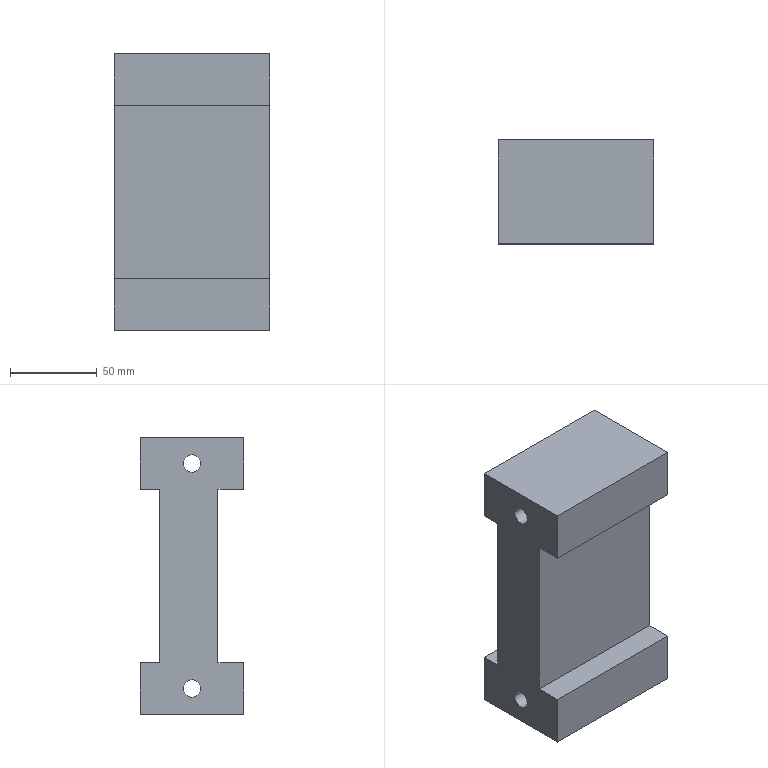Component | SolidWorks | TrackSupportBlock-2 | 1 solid | 18 faces | box 90 x 60 x 160 mm | volume 615863 mm3 | plane 14 | cylinder 4 | commonest cylinder face diameters 10 x4
build123d program:
from build123d import *

# Parameters (mm, degrees)
SKETCH1_W           = 60
SKETCH1_H           = 30
BOSS_EXTRUDE1_DEPTH = 90
SKETCH2_W           = 34
SKETCH2_H           = 90
BOSS_EXTRUDE2_DEPTH = 100
SKETCH3_W           = 60
SKETCH3_H           = 90
BOSS_EXTRUDE3_DEPTH = 30
SKETCH4_R           = 5
CUT_EXTRUDE1_DEPTH  = 90


with BuildPart() as part:
    # Sketch1 → Boss-Extrude1 (new body)
    with BuildSketch(Plane.XY):
        with Locations((91.434, -65)):
            Rectangle(SKETCH1_W, SKETCH1_H)
    extrude(amount=BOSS_EXTRUDE1_DEPTH)

    # Sketch2 → Boss-Extrude2 (add)
    with BuildSketch(Plane(origin=(0, -50, 0), x_dir=(1, 0, 0), z_dir=(0, 1, 0))):
        with Locations((93.434, -45)):
            Rectangle(SKETCH2_W, SKETCH2_H)
    extrude(amount=BOSS_EXTRUDE2_DEPTH)

    # Sketch3 → Boss-Extrude3 (add)
    with BuildSketch(Plane(origin=(0, 50, 0), x_dir=(1, 0, 0), z_dir=(0, 1, 0))):
        with Locations((91.434, -45)):
            Rectangle(SKETCH3_W, SKETCH3_H)
    extrude(amount=BOSS_EXTRUDE3_DEPTH)

    # Sketch4 → Cut-Extrude1 (cut)
    with BuildSketch(Plane.XY.offset(90)):
        with Locations((91.434, -65)):
            Circle(SKETCH4_R)
        with Locations((91.434, 65)):
            Circle(SKETCH4_R)
    extrude(amount=-CUT_EXTRUDE1_DEPTH, mode=Mode.SUBTRACT)


solid = part.part

# Placed as in the assembly
solid = solid.moved(Location((-195, -1.434, 0), (90, 90, 0)))
STEP:
#1=CARTESIAN_POINT('',(-4.134,3.346,2.559));
#2=VERTEX_POINT('',#1);
#3=CARTESIAN_POINT('',(-4.134,3.74,2.559));
#4=VERTEX_POINT('',#3);
#5=CARTESIAN_POINT('',(-4.134,3.543,2.559));
#6=DIRECTION('',(-1.,0.,0.));
#7=DIRECTION('',(0.,1.,0.));
#8=AXIS2_PLACEMENT_3D('',#5,#6,#7);
#9=CIRCLE('',#8,0.1969);
#10=EDGE_CURVE('',#2,#4,#9,.T.);
#11=ORIENTED_EDGE('',*,*,#10,.F.);
#12=CARTESIAN_POINT('',(-7.677,3.346,2.559));
#13=VERTEX_POINT('',#12);
#14=CARTESIAN_POINT('',(-4.134,3.346,2.559));
#15=DIRECTION('',(-1.,0.,0.));
#16=VECTOR('',#15,39.37);
#17=LINE('',#14,#16);
#18=EDGE_CURVE('',#2,#13,#17,.T.);
#19=ORIENTED_EDGE('',*,*,#18,.T.);
#20=CARTESIAN_POINT('',(-7.677,3.74,2.559));
#21=VERTEX_POINT('',#20);
#22=CARTESIAN_POINT('',(-7.677,3.543,2.559));
#23=DIRECTION('',(-1.,0.,0.));
#24=DIRECTION('',(0.,1.,0.));
#25=AXIS2_PLACEMENT_3D('',#22,#23,#24);
#26=CIRCLE('',#25,0.1969);
#27=EDGE_CURVE('',#13,#21,#26,.T.);
#28=ORIENTED_EDGE('',*,*,#27,.T.);
#29=CARTESIAN_POINT('',(-4.134,3.74,2.559));
#30=DIRECTION('',(-1.,0.,0.));
#31=VECTOR('',#30,39.37);
#32=LINE('',#29,#31);
#33=EDGE_CURVE('',#4,#21,#32,.T.);
#34=ORIENTED_EDGE('',*,*,#33,.F.);
#35=EDGE_LOOP('',(#11,#19,#28,#34));
#36=FACE_OUTER_BOUND('',#35,.T.);
#37=CARTESIAN_POINT('',(-4.134,3.543,2.559));
#38=DIRECTION('',(-1.,0.,0.));
#39=DIRECTION('',(0.,1.,0.));
#40=AXIS2_PLACEMENT_3D('',#37,#38,#39);
#41=CYLINDRICAL_SURFACE('',#40,0.1969);
#42=ADVANCED_FACE('',(#36),#41,.F.);
#43=CARTESIAN_POINT('',(-4.134,3.346,-2.559));
#44=VERTEX_POINT('',#43);
#45=CARTESIAN_POINT('',(-4.134,3.74,-2.559));
#46=VERTEX_POINT('',#45);
#47=CARTESIAN_POINT('',(-4.134,3.543,-2.559));
#48=DIRECTION('',(-1.,0.,0.));
#49=DIRECTION('',(0.,-1.,0.));
#50=AXIS2_PLACEMENT_3D('',#47,#48,#49);
#51=CIRCLE('',#50,0.1969);
#52=EDGE_CURVE('',#44,#46,#51,.T.);
#53=ORIENTED_EDGE('',*,*,#52,.F.);
#54=CARTESIAN_POINT('',(-7.677,3.346,-2.559));
#55=VERTEX_POINT('',#54);
#56=CARTESIAN_POINT('',(-4.134,3.346,-2.559));
#57=DIRECTION('',(-1.,0.,0.));
#58=VECTOR('',#57,39.37);
#59=LINE('',#56,#58);
#60=EDGE_CURVE('',#44,#55,#59,.T.);
#61=ORIENTED_EDGE('',*,*,#60,.T.);
#62=CARTESIAN_POINT('',(-7.677,3.74,-2.559));
#63=VERTEX_POINT('',#62);
#64=CARTESIAN_POINT('',(-7.677,3.543,-2.559));
#65=DIRECTION('',(-1.,0.,0.));
#66=DIRECTION('',(0.,-1.,0.));
#67=AXIS2_PLACEMENT_3D('',#64,#65,#66);
#68=CIRCLE('',#67,0.1969);
#69=EDGE_CURVE('',#55,#63,#68,.T.);
#70=ORIENTED_EDGE('',*,*,#69,.T.);
#71=CARTESIAN_POINT('',(-4.134,3.74,-2.559));
#72=DIRECTION('',(-1.,0.,0.));
#73=VECTOR('',#72,39.37);
#74=LINE('',#71,#73);
#75=EDGE_CURVE('',#46,#63,#74,.T.);
#76=ORIENTED_EDGE('',*,*,#75,.F.);
#77=EDGE_LOOP('',(#53,#61,#70,#76));
#78=FACE_OUTER_BOUND('',#77,.T.);
#79=CARTESIAN_POINT('',(-4.134,3.543,-2.559));
#80=DIRECTION('',(-1.,0.,0.));
#81=DIRECTION('',(0.,1.,0.));
#82=AXIS2_PLACEMENT_3D('',#79,#80,#81);
#83=CYLINDRICAL_SURFACE('',#82,0.1969);
#84=ADVANCED_FACE('',(#78),#83,.F.);
#85=CARTESIAN_POINT('',(-7.677,4.291,1.969));
#86=VERTEX_POINT('',#85);
#87=CARTESIAN_POINT('',(-4.134,4.291,1.969));
#88=VERTEX_POINT('',#87);
#89=CARTESIAN_POINT('',(-4.134,4.291,1.969));
#90=DIRECTION('',(1.,0.,0.));
#91=VECTOR('',#90,39.37);
#92=LINE('',#89,#91);
#93=EDGE_CURVE('',#86,#88,#92,.T.);
#94=ORIENTED_EDGE('',*,*,#93,.F.);
#95=CARTESIAN_POINT('',(-7.677,4.724,1.969));
#96=VERTEX_POINT('',#95);
#97=CARTESIAN_POINT('',(-7.677,4.724,1.969));
#98=DIRECTION('',(0.,-1.,0.));
#99=VECTOR('',#98,39.37);
#100=LINE('',#97,#99);
#101=EDGE_CURVE('',#96,#86,#100,.T.);
#102=ORIENTED_EDGE('',*,*,#101,.F.);
#103=CARTESIAN_POINT('',(-4.134,4.724,1.969));
#104=VERTEX_POINT('',#103);
#105=CARTESIAN_POINT('',(-7.677,4.724,1.969));
#106=DIRECTION('',(1.,0.,0.));
#107=VECTOR('',#106,39.37);
#108=LINE('',#105,#107);
#109=EDGE_CURVE('',#96,#104,#108,.T.);
#110=ORIENTED_EDGE('',*,*,#109,.T.);
#111=CARTESIAN_POINT('',(-4.134,4.724,1.969));
#112=DIRECTION('',(0.,-1.,0.));
#113=VECTOR('',#112,39.37);
#114=LINE('',#111,#113);
#115=EDGE_CURVE('',#104,#88,#114,.T.);
#116=ORIENTED_EDGE('',*,*,#115,.T.);
#117=EDGE_LOOP('',(#94,#102,#110,#116));
#118=FACE_OUTER_BOUND('',#117,.T.);
#119=CARTESIAN_POINT('',(-7.677,4.724,1.969));
#120=DIRECTION('',(0.,0.,1.));
#121=DIRECTION('',(1.,0.,0.));
#122=AXIS2_PLACEMENT_3D('',#119,#120,#121);
#123=PLANE('',#122);
#124=ADVANCED_FACE('',(#118),#123,.F.);
#125=CARTESIAN_POINT('',(-4.134,2.953,1.969));
#126=VERTEX_POINT('',#125);
#127=CARTESIAN_POINT('',(-7.677,2.953,1.969));
#128=VERTEX_POINT('',#127);
#129=CARTESIAN_POINT('',(-4.134,2.953,1.969));
#130=DIRECTION('',(-1.,0.,0.));
#131=VECTOR('',#130,39.37);
#132=LINE('',#129,#131);
#133=EDGE_CURVE('',#126,#128,#132,.T.);
#134=ORIENTED_EDGE('',*,*,#133,.F.);
#135=CARTESIAN_POINT('',(-4.134,2.362,1.969));
#136=VERTEX_POINT('',#135);
#137=CARTESIAN_POINT('',(-4.134,4.724,1.969));
#138=DIRECTION('',(0.,-1.,0.));
#139=VECTOR('',#138,39.37);
#140=LINE('',#137,#139);
#141=EDGE_CURVE('',#126,#136,#140,.T.);
#142=ORIENTED_EDGE('',*,*,#141,.T.);
#143=CARTESIAN_POINT('',(-7.677,2.362,1.969));
#144=VERTEX_POINT('',#143);
#145=CARTESIAN_POINT('',(-7.677,2.362,1.969));
#146=DIRECTION('',(1.,0.,0.));
#147=VECTOR('',#146,39.37);
#148=LINE('',#145,#147);
#149=EDGE_CURVE('',#144,#136,#148,.T.);
#150=ORIENTED_EDGE('',*,*,#149,.F.);
#151=CARTESIAN_POINT('',(-7.677,4.724,1.969));
#152=DIRECTION('',(0.,-1.,0.));
#153=VECTOR('',#152,39.37);
#154=LINE('',#151,#153);
#155=EDGE_CURVE('',#128,#144,#154,.T.);
#156=ORIENTED_EDGE('',*,*,#155,.F.);
#157=EDGE_LOOP('',(#134,#142,#150,#156));
#158=FACE_OUTER_BOUND('',#157,.T.);
#159=CARTESIAN_POINT('',(-7.677,4.724,1.969));
#160=DIRECTION('',(0.,0.,1.));
#161=DIRECTION('',(1.,0.,0.));
#162=AXIS2_PLACEMENT_3D('',#159,#160,#161);
#163=PLANE('',#162);
#164=ADVANCED_FACE('',(#158),#163,.F.);
#165=CARTESIAN_POINT('',(-4.134,4.724,3.15));
#166=VERTEX_POINT('',#165);
#167=CARTESIAN_POINT('',(-4.134,4.724,1.969));
#168=DIRECTION('',(0.,0.,-1.));
#169=VECTOR('',#168,39.37);
#170=LINE('',#167,#169);
#171=EDGE_CURVE('',#166,#104,#170,.T.);
#172=ORIENTED_EDGE('',*,*,#171,.T.);
#173=ORIENTED_EDGE('',*,*,#109,.F.);
#174=CARTESIAN_POINT('',(-7.677,4.724,3.15));
#175=VERTEX_POINT('',#174);
#176=CARTESIAN_POINT('',(-7.677,4.724,1.969));
#177=DIRECTION('',(0.,0.,-1.));
#178=VECTOR('',#177,39.37);
#179=LINE('',#176,#178);
#180=EDGE_CURVE('',#175,#96,#179,.T.);
#181=ORIENTED_EDGE('',*,*,#180,.F.);
#182=CARTESIAN_POINT('',(-7.677,4.724,3.15));
#183=DIRECTION('',(1.,0.,0.));
#184=VECTOR('',#183,39.37);
#185=LINE('',#182,#184);
#186=EDGE_CURVE('',#175,#166,#185,.T.);
#187=ORIENTED_EDGE('',*,*,#186,.T.);
#188=EDGE_LOOP('',(#172,#173,#181,#187));
#189=FACE_OUTER_BOUND('',#188,.T.);
#190=CARTESIAN_POINT('',(-7.677,4.724,1.969));
#191=DIRECTION('',(0.,-1.,0.));
#192=DIRECTION('',(-1.,0.,0.));
#193=AXIS2_PLACEMENT_3D('',#190,#191,#192);
#194=PLANE('',#193);
#195=ADVANCED_FACE('',(#189),#194,.F.);
#196=CARTESIAN_POINT('',(-4.134,2.362,3.15));
#197=VERTEX_POINT('',#196);
#198=CARTESIAN_POINT('',(-4.134,2.362,1.969));
#199=DIRECTION('',(0.,0.,1.));
#200=VECTOR('',#199,39.37);
#201=LINE('',#198,#200);
#202=EDGE_CURVE('',#136,#197,#201,.T.);
#203=ORIENTED_EDGE('',*,*,#202,.T.);
#204=CARTESIAN_POINT('',(-7.677,2.362,3.15));
#205=VERTEX_POINT('',#204);
#206=CARTESIAN_POINT('',(-7.677,2.362,3.15));
#207=DIRECTION('',(1.,0.,0.));
#208=VECTOR('',#207,39.37);
#209=LINE('',#206,#208);
#210=EDGE_CURVE('',#205,#197,#209,.T.);
#211=ORIENTED_EDGE('',*,*,#210,.F.);
#212=CARTESIAN_POINT('',(-7.677,2.362,1.969));
#213=DIRECTION('',(0.,0.,1.));
#214=VECTOR('',#213,39.37);
#215=LINE('',#212,#214);
#216=EDGE_CURVE('',#144,#205,#215,.T.);
#217=ORIENTED_EDGE('',*,*,#216,.F.);
#218=ORIENTED_EDGE('',*,*,#149,.T.);
#219=EDGE_LOOP('',(#203,#211,#217,#218));
#220=FACE_OUTER_BOUND('',#219,.T.);
#221=CARTESIAN_POINT('',(-7.677,2.362,1.969));
#222=DIRECTION('',(0.,1.,-0.));
#223=DIRECTION('',(0.,-0.,-1.));
#224=AXIS2_PLACEMENT_3D('',#221,#222,#223);
#225=PLANE('',#224);
#226=ADVANCED_FACE('',(#220),#225,.F.);
#227=CARTESIAN_POINT('',(-4.134,4.724,3.15));
#228=DIRECTION('',(0.,1.,0.));
#229=VECTOR('',#228,39.37);
#230=LINE('',#227,#229);
#231=EDGE_CURVE('',#197,#166,#230,.T.);
#232=ORIENTED_EDGE('',*,*,#231,.T.);
#233=ORIENTED_EDGE('',*,*,#186,.F.);
#234=CARTESIAN_POINT('',(-7.677,4.724,3.15));
#235=DIRECTION('',(0.,1.,0.));
#236=VECTOR('',#235,39.37);
#237=LINE('',#234,#236);
#238=EDGE_CURVE('',#205,#175,#237,.T.);
#239=ORIENTED_EDGE('',*,*,#238,.F.);
#240=ORIENTED_EDGE('',*,*,#210,.T.);
#241=EDGE_LOOP('',(#232,#233,#239,#240));
#242=FACE_OUTER_BOUND('',#241,.T.);
#243=CARTESIAN_POINT('',(-7.677,4.724,3.15));
#244=DIRECTION('',(0.,0.,-1.));
#245=DIRECTION('',(-1.,0.,0.));
#246=AXIS2_PLACEMENT_3D('',#243,#244,#245);
#247=PLANE('',#246);
#248=ADVANCED_FACE('',(#242),#247,.F.);
#249=CARTESIAN_POINT('',(-7.677,3.543,2.559));
#250=DIRECTION('',(-1.,0.,0.));
#251=DIRECTION('',(0.,1.,0.));
#252=AXIS2_PLACEMENT_3D('',#249,#250,#251);
#253=CIRCLE('',#252,0.1969);
#254=EDGE_CURVE('',#21,#13,#253,.T.);
#255=ORIENTED_EDGE('',*,*,#254,.F.);
#256=ORIENTED_EDGE('',*,*,#27,.F.);
#257=EDGE_LOOP('',(#255,#256));
#258=FACE_BOUND('',#257,.T.);
#259=CARTESIAN_POINT('',(-7.677,3.543,-2.559));
#260=DIRECTION('',(-1.,0.,0.));
#261=DIRECTION('',(0.,-1.,0.));
#262=AXIS2_PLACEMENT_3D('',#259,#260,#261);
#263=CIRCLE('',#262,0.1969);
#264=EDGE_CURVE('',#63,#55,#263,.T.);
#265=ORIENTED_EDGE('',*,*,#264,.F.);
#266=ORIENTED_EDGE('',*,*,#69,.F.);
#267=EDGE_LOOP('',(#265,#266));
#268=FACE_BOUND('',#267,.T.);
#269=ORIENTED_EDGE('',*,*,#180,.T.);
#270=ORIENTED_EDGE('',*,*,#101,.T.);
#271=CARTESIAN_POINT('',(-7.677,4.291,-1.969));
#272=VERTEX_POINT('',#271);
#273=CARTESIAN_POINT('',(-7.677,4.291,-1.969));
#274=DIRECTION('',(0.,0.,1.));
#275=VECTOR('',#274,39.37);
#276=LINE('',#273,#275);
#277=EDGE_CURVE('',#272,#86,#276,.T.);
#278=ORIENTED_EDGE('',*,*,#277,.F.);
#279=CARTESIAN_POINT('',(-7.677,4.724,-1.969));
#280=VERTEX_POINT('',#279);
#281=CARTESIAN_POINT('',(-7.677,4.724,-1.969));
#282=DIRECTION('',(0.,1.,0.));
#283=VECTOR('',#282,39.37);
#284=LINE('',#281,#283);
#285=EDGE_CURVE('',#272,#280,#284,.T.);
#286=ORIENTED_EDGE('',*,*,#285,.T.);
#287=CARTESIAN_POINT('',(-7.677,4.724,-3.15));
#288=VERTEX_POINT('',#287);
#289=CARTESIAN_POINT('',(-7.677,4.724,-3.15));
#290=DIRECTION('',(0.,0.,1.));
#291=VECTOR('',#290,39.37);
#292=LINE('',#289,#291);
#293=EDGE_CURVE('',#288,#280,#292,.T.);
#294=ORIENTED_EDGE('',*,*,#293,.F.);
#295=CARTESIAN_POINT('',(-7.677,2.362,-3.15));
#296=VERTEX_POINT('',#295);
#297=CARTESIAN_POINT('',(-7.677,4.724,-3.15));
#298=DIRECTION('',(0.,1.,0.));
#299=VECTOR('',#298,39.37);
#300=LINE('',#297,#299);
#301=EDGE_CURVE('',#296,#288,#300,.T.);
#302=ORIENTED_EDGE('',*,*,#301,.F.);
#303=CARTESIAN_POINT('',(-7.677,2.362,-1.969));
#304=VERTEX_POINT('',#303);
#305=CARTESIAN_POINT('',(-7.677,2.362,-3.15));
#306=DIRECTION('',(0.,0.,1.));
#307=VECTOR('',#306,39.37);
#308=LINE('',#305,#307);
#309=EDGE_CURVE('',#296,#304,#308,.T.);
#310=ORIENTED_EDGE('',*,*,#309,.T.);
#311=CARTESIAN_POINT('',(-7.677,2.953,-1.969));
#312=VERTEX_POINT('',#311);
#313=CARTESIAN_POINT('',(-7.677,4.724,-1.969));
#314=DIRECTION('',(0.,1.,0.));
#315=VECTOR('',#314,39.37);
#316=LINE('',#313,#315);
#317=EDGE_CURVE('',#304,#312,#316,.T.);
#318=ORIENTED_EDGE('',*,*,#317,.T.);
#319=CARTESIAN_POINT('',(-7.677,2.953,-1.969));
#320=DIRECTION('',(0.,0.,1.));
#321=VECTOR('',#320,39.37);
#322=LINE('',#319,#321);
#323=EDGE_CURVE('',#312,#128,#322,.T.);
#324=ORIENTED_EDGE('',*,*,#323,.T.);
#325=ORIENTED_EDGE('',*,*,#155,.T.);
#326=ORIENTED_EDGE('',*,*,#216,.T.);
#327=ORIENTED_EDGE('',*,*,#238,.T.);
#328=EDGE_LOOP('',(#269,#270,#278,#286,#294,#302,#310,#318,#324,#325,#326,#327));
#329=FACE_OUTER_BOUND('',#328,.T.);
#330=CARTESIAN_POINT('',(-7.677,-0.05646,-0.));
#331=DIRECTION('',(1.,0.,0.));
#332=DIRECTION('',(0.,-1.,0.));
#333=AXIS2_PLACEMENT_3D('',#330,#331,#332);
#334=PLANE('',#333);
#335=ADVANCED_FACE('',(#258,#268,#329),#334,.F.);
#336=CARTESIAN_POINT('',(-4.134,3.543,2.559));
#337=DIRECTION('',(-1.,0.,0.));
#338=DIRECTION('',(0.,1.,0.));
#339=AXIS2_PLACEMENT_3D('',#336,#337,#338);
#340=CIRCLE('',#339,0.1969);
#341=EDGE_CURVE('',#4,#2,#340,.T.);
#342=ORIENTED_EDGE('',*,*,#341,.T.);
#343=ORIENTED_EDGE('',*,*,#10,.T.);
#344=EDGE_LOOP('',(#342,#343));
#345=FACE_BOUND('',#344,.T.);
#346=CARTESIAN_POINT('',(-4.134,3.543,-2.559));
#347=DIRECTION('',(-1.,0.,0.));
#348=DIRECTION('',(0.,-1.,0.));
#349=AXIS2_PLACEMENT_3D('',#346,#347,#348);
#350=CIRCLE('',#349,0.1969);
#351=EDGE_CURVE('',#46,#44,#350,.T.);
#352=ORIENTED_EDGE('',*,*,#351,.T.);
#353=ORIENTED_EDGE('',*,*,#52,.T.);
#354=EDGE_LOOP('',(#352,#353));
#355=FACE_BOUND('',#354,.T.);
#356=ORIENTED_EDGE('',*,*,#171,.F.);
#357=ORIENTED_EDGE('',*,*,#231,.F.);
#358=ORIENTED_EDGE('',*,*,#202,.F.);
#359=ORIENTED_EDGE('',*,*,#141,.F.);
#360=CARTESIAN_POINT('',(-4.134,2.953,-1.969));
#361=VERTEX_POINT('',#360);
#362=CARTESIAN_POINT('',(-4.134,2.953,-1.969));
#363=DIRECTION('',(0.,0.,1.));
#364=VECTOR('',#363,39.37);
#365=LINE('',#362,#364);
#366=EDGE_CURVE('',#361,#126,#365,.T.);
#367=ORIENTED_EDGE('',*,*,#366,.F.);
#368=CARTESIAN_POINT('',(-4.134,2.362,-1.969));
#369=VERTEX_POINT('',#368);
#370=CARTESIAN_POINT('',(-4.134,4.724,-1.969));
#371=DIRECTION('',(0.,-1.,0.));
#372=VECTOR('',#371,39.37);
#373=LINE('',#370,#372);
#374=EDGE_CURVE('',#361,#369,#373,.T.);
#375=ORIENTED_EDGE('',*,*,#374,.T.);
#376=CARTESIAN_POINT('',(-4.134,2.362,-3.15));
#377=VERTEX_POINT('',#376);
#378=CARTESIAN_POINT('',(-4.134,2.362,-3.15));
#379=DIRECTION('',(0.,0.,1.));
#380=VECTOR('',#379,39.37);
#381=LINE('',#378,#380);
#382=EDGE_CURVE('',#377,#369,#381,.T.);
#383=ORIENTED_EDGE('',*,*,#382,.F.);
#384=CARTESIAN_POINT('',(-4.134,4.724,-3.15));
#385=VERTEX_POINT('',#384);
#386=CARTESIAN_POINT('',(-4.134,4.724,-3.15));
#387=DIRECTION('',(0.,-1.,0.));
#388=VECTOR('',#387,39.37);
#389=LINE('',#386,#388);
#390=EDGE_CURVE('',#385,#377,#389,.T.);
#391=ORIENTED_EDGE('',*,*,#390,.F.);
#392=CARTESIAN_POINT('',(-4.134,4.724,-1.969));
#393=VERTEX_POINT('',#392);
#394=CARTESIAN_POINT('',(-4.134,4.724,-3.15));
#395=DIRECTION('',(0.,0.,1.));
#396=VECTOR('',#395,39.37);
#397=LINE('',#394,#396);
#398=EDGE_CURVE('',#385,#393,#397,.T.);
#399=ORIENTED_EDGE('',*,*,#398,.T.);
#400=CARTESIAN_POINT('',(-4.134,4.291,-1.969));
#401=VERTEX_POINT('',#400);
#402=CARTESIAN_POINT('',(-4.134,4.724,-1.969));
#403=DIRECTION('',(0.,-1.,0.));
#404=VECTOR('',#403,39.37);
#405=LINE('',#402,#404);
#406=EDGE_CURVE('',#393,#401,#405,.T.);
#407=ORIENTED_EDGE('',*,*,#406,.T.);
#408=CARTESIAN_POINT('',(-4.134,4.291,-1.969));
#409=DIRECTION('',(0.,0.,1.));
#410=VECTOR('',#409,39.37);
#411=LINE('',#408,#410);
#412=EDGE_CURVE('',#401,#88,#411,.T.);
#413=ORIENTED_EDGE('',*,*,#412,.T.);
#414=ORIENTED_EDGE('',*,*,#115,.F.);
#415=EDGE_LOOP('',(#356,#357,#358,#359,#367,#375,#383,#391,#399,#407,#413,#414));
#416=FACE_OUTER_BOUND('',#415,.T.);
#417=CARTESIAN_POINT('',(-4.134,-0.05646,-0.));
#418=DIRECTION('',(1.,0.,0.));
#419=DIRECTION('',(0.,-1.,0.));
#420=AXIS2_PLACEMENT_3D('',#417,#418,#419);
#421=PLANE('',#420);
#422=ADVANCED_FACE('',(#345,#355,#416),#421,.T.);
#423=ORIENTED_EDGE('',*,*,#93,.T.);
#424=ORIENTED_EDGE('',*,*,#412,.F.);
#425=CARTESIAN_POINT('',(-4.134,4.291,-1.969));
#426=DIRECTION('',(1.,0.,0.));
#427=VECTOR('',#426,39.37);
#428=LINE('',#425,#427);
#429=EDGE_CURVE('',#272,#401,#428,.T.);
#430=ORIENTED_EDGE('',*,*,#429,.F.);
#431=ORIENTED_EDGE('',*,*,#277,.T.);
#432=EDGE_LOOP('',(#423,#424,#430,#431));
#433=FACE_OUTER_BOUND('',#432,.T.);
#434=CARTESIAN_POINT('',(-4.134,4.291,-1.969));
#435=DIRECTION('',(0.,-1.,0.));
#436=DIRECTION('',(-1.,0.,0.));
#437=AXIS2_PLACEMENT_3D('',#434,#435,#436);
#438=PLANE('',#437);
#439=ADVANCED_FACE('',(#433),#438,.F.);
#440=ORIENTED_EDGE('',*,*,#133,.T.);
#441=ORIENTED_EDGE('',*,*,#323,.F.);
#442=CARTESIAN_POINT('',(-4.134,2.953,-1.969));
#443=DIRECTION('',(-1.,0.,0.));
#444=VECTOR('',#443,39.37);
#445=LINE('',#442,#444);
#446=EDGE_CURVE('',#361,#312,#445,.T.);
#447=ORIENTED_EDGE('',*,*,#446,.F.);
#448=ORIENTED_EDGE('',*,*,#366,.T.);
#449=EDGE_LOOP('',(#440,#441,#447,#448));
#450=FACE_OUTER_BOUND('',#449,.T.);
#451=CARTESIAN_POINT('',(-4.134,2.953,-1.969));
#452=DIRECTION('',(0.,1.,0.));
#453=DIRECTION('',(1.,0.,0.));
#454=AXIS2_PLACEMENT_3D('',#451,#452,#453);
#455=PLANE('',#454);
#456=ADVANCED_FACE('',(#450),#455,.F.);
#457=ORIENTED_EDGE('',*,*,#285,.F.);
#458=ORIENTED_EDGE('',*,*,#429,.T.);
#459=ORIENTED_EDGE('',*,*,#406,.F.);
#460=CARTESIAN_POINT('',(-4.134,4.724,-1.969));
#461=DIRECTION('',(1.,0.,0.));
#462=VECTOR('',#461,39.37);
#463=LINE('',#460,#462);
#464=EDGE_CURVE('',#280,#393,#463,.T.);
#465=ORIENTED_EDGE('',*,*,#464,.F.);
#466=EDGE_LOOP('',(#457,#458,#459,#465));
#467=FACE_OUTER_BOUND('',#466,.T.);
#468=CARTESIAN_POINT('',(-4.134,-0.05646,-1.969));
#469=DIRECTION('',(0.,0.,1.));
#470=DIRECTION('',(1.,0.,0.));
#471=AXIS2_PLACEMENT_3D('',#468,#469,#470);
#472=PLANE('',#471);
#473=ADVANCED_FACE('',(#467),#472,.T.);
#474=ORIENTED_EDGE('',*,*,#464,.T.);
#475=ORIENTED_EDGE('',*,*,#398,.F.);
#476=CARTESIAN_POINT('',(-4.134,4.724,-3.15));
#477=DIRECTION('',(1.,0.,0.));
#478=VECTOR('',#477,39.37);
#479=LINE('',#476,#478);
#480=EDGE_CURVE('',#288,#385,#479,.T.);
#481=ORIENTED_EDGE('',*,*,#480,.F.);
#482=ORIENTED_EDGE('',*,*,#293,.T.);
#483=EDGE_LOOP('',(#474,#475,#481,#482));
#484=FACE_OUTER_BOUND('',#483,.T.);
#485=CARTESIAN_POINT('',(-4.134,4.724,-3.15));
#486=DIRECTION('',(0.,-1.,0.));
#487=DIRECTION('',(-1.,0.,0.));
#488=AXIS2_PLACEMENT_3D('',#485,#486,#487);
#489=PLANE('',#488);
#490=ADVANCED_FACE('',(#484),#489,.F.);
#491=CARTESIAN_POINT('',(-4.134,2.362,-1.969));
#492=DIRECTION('',(-1.,0.,0.));
#493=VECTOR('',#492,39.37);
#494=LINE('',#491,#493);
#495=EDGE_CURVE('',#369,#304,#494,.T.);
#496=ORIENTED_EDGE('',*,*,#495,.T.);
#497=ORIENTED_EDGE('',*,*,#309,.F.);
#498=CARTESIAN_POINT('',(-4.134,2.362,-3.15));
#499=DIRECTION('',(-1.,0.,0.));
#500=VECTOR('',#499,39.37);
#501=LINE('',#498,#500);
#502=EDGE_CURVE('',#377,#296,#501,.T.);
#503=ORIENTED_EDGE('',*,*,#502,.F.);
#504=ORIENTED_EDGE('',*,*,#382,.T.);
#505=EDGE_LOOP('',(#496,#497,#503,#504));
#506=FACE_OUTER_BOUND('',#505,.T.);
#507=CARTESIAN_POINT('',(-4.134,2.362,-3.15));
#508=DIRECTION('',(0.,1.,0.));
#509=DIRECTION('',(1.,0.,0.));
#510=AXIS2_PLACEMENT_3D('',#507,#508,#509);
#511=PLANE('',#510);
#512=ADVANCED_FACE('',(#506),#511,.F.);
#513=ORIENTED_EDGE('',*,*,#480,.T.);
#514=ORIENTED_EDGE('',*,*,#390,.T.);
#515=ORIENTED_EDGE('',*,*,#502,.T.);
#516=ORIENTED_EDGE('',*,*,#301,.T.);
#517=EDGE_LOOP('',(#513,#514,#515,#516));
#518=FACE_OUTER_BOUND('',#517,.T.);
#519=CARTESIAN_POINT('',(-4.134,-0.05646,-3.15));
#520=DIRECTION('',(0.,0.,1.));
#521=DIRECTION('',(1.,0.,0.));
#522=AXIS2_PLACEMENT_3D('',#519,#520,#521);
#523=PLANE('',#522);
#524=ADVANCED_FACE('',(#518),#523,.F.);
#525=ORIENTED_EDGE('',*,*,#374,.F.);
#526=ORIENTED_EDGE('',*,*,#446,.T.);
#527=ORIENTED_EDGE('',*,*,#317,.F.);
#528=ORIENTED_EDGE('',*,*,#495,.F.);
#529=EDGE_LOOP('',(#525,#526,#527,#528));
#530=FACE_OUTER_BOUND('',#529,.T.);
#531=CARTESIAN_POINT('',(-4.134,-0.05646,-1.969));
#532=DIRECTION('',(0.,0.,1.));
#533=DIRECTION('',(1.,0.,0.));
#534=AXIS2_PLACEMENT_3D('',#531,#532,#533);
#535=PLANE('',#534);
#536=ADVANCED_FACE('',(#530),#535,.T.);
#537=ORIENTED_EDGE('',*,*,#60,.F.);
#538=ORIENTED_EDGE('',*,*,#351,.F.);
#539=ORIENTED_EDGE('',*,*,#75,.T.);
#540=ORIENTED_EDGE('',*,*,#264,.T.);
#541=EDGE_LOOP('',(#537,#538,#539,#540));
#542=FACE_OUTER_BOUND('',#541,.T.);
#543=CARTESIAN_POINT('',(-4.134,3.543,-2.559));
#544=DIRECTION('',(-1.,0.,0.));
#545=DIRECTION('',(0.,1.,0.));
#546=AXIS2_PLACEMENT_3D('',#543,#544,#545);
#547=CYLINDRICAL_SURFACE('',#546,0.1969);
#548=ADVANCED_FACE('',(#542),#547,.F.);
#549=ORIENTED_EDGE('',*,*,#18,.F.);
#550=ORIENTED_EDGE('',*,*,#341,.F.);
#551=ORIENTED_EDGE('',*,*,#33,.T.);
#552=ORIENTED_EDGE('',*,*,#254,.T.);
#553=EDGE_LOOP('',(#549,#550,#551,#552));
#554=FACE_OUTER_BOUND('',#553,.T.);
#555=CARTESIAN_POINT('',(-4.134,3.543,2.559));
#556=DIRECTION('',(-1.,0.,0.));
#557=DIRECTION('',(0.,1.,0.));
#558=AXIS2_PLACEMENT_3D('',#555,#556,#557);
#559=CYLINDRICAL_SURFACE('',#558,0.1969);
#560=ADVANCED_FACE('',(#554),#559,.F.);
#561=CLOSED_SHELL('',(#42,#84,#124,#164,#195,#226,#248,#335,#422,#439,#456,#473,#490,#512,#524,#536,#548,#560));
#562=MANIFOLD_SOLID_BREP('',#561);
#563=CARTESIAN_POINT('',(0.,0.,0.));
#564=DIRECTION('',(0.,0.,1.));
#565=DIRECTION('',(1.,0.,0.));
#566=AXIS2_PLACEMENT_3D('',#563,#564,#565);
#567=(LENGTH_UNIT()NAMED_UNIT(*)SI_UNIT($,.METRE.));
#568=LENGTH_MEASURE_WITH_UNIT(LENGTH_MEASURE(0.0254),#567);
#569=DIMENSIONAL_EXPONENTS(1.,0.,0.,0.,0.,0.,0.);
#570=(CONVERSION_BASED_UNIT('',#568)LENGTH_UNIT()NAMED_UNIT(#569));
#571=UNCERTAINTY_MEASURE_WITH_UNIT(LENGTH_MEASURE(0.00001),#570,'','');
#572=(NAMED_UNIT(*)PLANE_ANGLE_UNIT()SI_UNIT($,.RADIAN.));
#573=(NAMED_UNIT(*)SI_UNIT($,.STERADIAN.)SOLID_ANGLE_UNIT());
#574=(GEOMETRIC_REPRESENTATION_CONTEXT(3)GLOBAL_UNCERTAINTY_ASSIGNED_CONTEXT((#571))GLOBAL_UNIT_ASSIGNED_CONTEXT((#570,#572,#573))REPRESENTATION_CONTEXT('',''));
#575=ADVANCED_BREP_SHAPE_REPRESENTATION('',(#562,#566),#574);
#576=COLOUR_RGB('',0.7922,0.8196,0.9333);
#577=FILL_AREA_STYLE_COLOUR('',#576);
#578=FILL_AREA_STYLE('',(#577));
#579=SURFACE_STYLE_FILL_AREA(#578);
#580=SURFACE_SIDE_STYLE('',(#579));
#581=SURFACE_STYLE_USAGE(.BOTH.,#580);
#582=PRESENTATION_STYLE_ASSIGNMENT((#581));
#583=STYLED_ITEM('',(#582),#562);
#584=(LENGTH_UNIT()NAMED_UNIT(*)SI_UNIT($,.METRE.));
#585=LENGTH_MEASURE_WITH_UNIT(LENGTH_MEASURE(0.0254),#584);
#586=DIMENSIONAL_EXPONENTS(1.,0.,0.,0.,0.,0.,0.);
#587=(CONVERSION_BASED_UNIT('',#585)LENGTH_UNIT()NAMED_UNIT(#586));
#588=UNCERTAINTY_MEASURE_WITH_UNIT(LENGTH_MEASURE(0.00001),#587,'','');
#589=(NAMED_UNIT(*)PLANE_ANGLE_UNIT()SI_UNIT($,.RADIAN.));
#590=(NAMED_UNIT(*)SI_UNIT($,.STERADIAN.)SOLID_ANGLE_UNIT());
#591=(GEOMETRIC_REPRESENTATION_CONTEXT(3)GLOBAL_UNCERTAINTY_ASSIGNED_CONTEXT((#588))GLOBAL_UNIT_ASSIGNED_CONTEXT((#587,#589,#590))REPRESENTATION_CONTEXT('',''));
#592=MECHANICAL_DESIGN_GEOMETRIC_PRESENTATION_REPRESENTATION('',(#583),#591);
#593=PRESENTATION_LAYER_ASSIGNMENT('','',(#583));